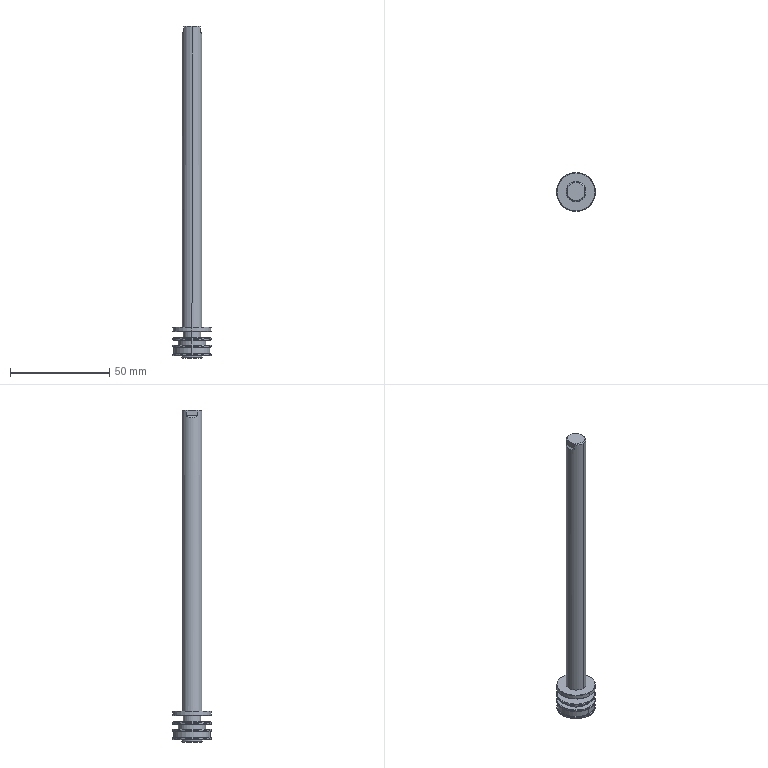Component | SolidWorks | TR-20x75-S-GN-1 (0)-3_TR-20x75-SCylinderRod-1 | 1 solid | 53 faces | volume 15105 mm3 | cylinder 18 | cone 17 | plane 14 | spline 4 | commonest cylinder face diameters 19.6 x8 10 x2 8.8 x2 14 x2 18.4 x2 10.6 x2